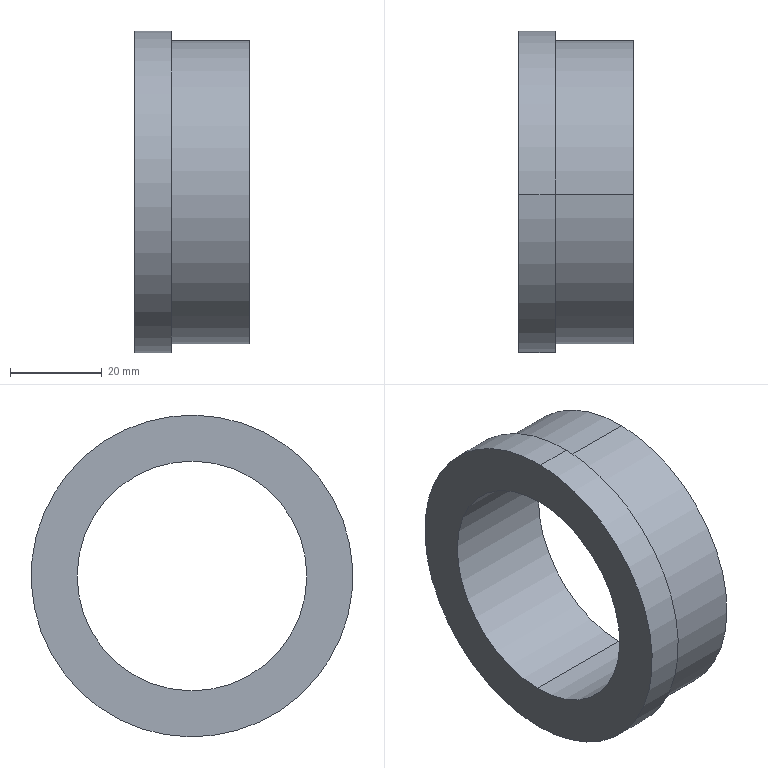Component | SolidWorks | 216InnerTubeAssembly-1_GuideSleeve-1 | 1 solid | 9 faces | box 25 x 70 x 70 mm | volume 39861 mm3 | cylinder 6 | plane 3 | commonest cylinder face diameters 50 x2 66 x2 70 x2 | material Alloy Steel
build123d program:
from build123d import *


with BuildPart() as part:
    # Model → Revolve1 (revolve)
    with BuildSketch(Plane.XY, mode=Mode.PRIVATE) as revolve1_sk:
        Polygon((-25, 35), (-17, 35), (-17, 33), (0, 33), (0, 25), (-25, 25), align=None)
    revolve(revolve1_sk.sketch.rotate(Axis((11.515, 0, 0), (-1, 0, 0)), 90), axis=Axis((11.515, 0, 0), (-1, 0, 0)))


solid = part.part

# Placed as in the assembly
solid = solid.moved(Location((527.091, 0, 0), (0, 0, 0)))
STEP:
#1=COLOUR_RGB('',0.7922,0.8196,0.9333);
#2=FILL_AREA_STYLE_COLOUR('',#1);
#3=FILL_AREA_STYLE('',(#2));
#4=SURFACE_STYLE_FILL_AREA(#3);
#5=SURFACE_SIDE_STYLE('',(#4));
#6=SURFACE_STYLE_USAGE(.BOTH.,#5);
#7=PRESENTATION_STYLE_ASSIGNMENT((#6));
#8=CARTESIAN_POINT('',(19.767,-0.01767,0.9841));
#9=VERTEX_POINT('',#8);
#10=CARTESIAN_POINT('',(19.767,0.01767,-0.9841));
#11=VERTEX_POINT('',#10);
#12=CARTESIAN_POINT('',(19.767,-0.,0.));
#13=DIRECTION('',(1.,0.,-0.));
#14=DIRECTION('',(0.,0.01796,-0.9998));
#15=AXIS2_PLACEMENT_3D('',#12,#13,#14);
#16=CIRCLE('',#15,0.9843);
#17=EDGE_CURVE('',#9,#11,#16,.T.);
#18=ORIENTED_EDGE('',*,*,#17,.F.);
#19=CARTESIAN_POINT('',(20.752,-0.01767,0.9841));
#20=VERTEX_POINT('',#19);
#21=CARTESIAN_POINT('',(21.205,-0.01767,0.9841));
#22=DIRECTION('',(1.,0.,-0.));
#23=VECTOR('',#22,39.37);
#24=LINE('',#21,#23);
#25=EDGE_CURVE('',#9,#20,#24,.T.);
#26=ORIENTED_EDGE('',*,*,#25,.T.);
#27=CARTESIAN_POINT('',(20.752,0.01767,-0.9841));
#28=VERTEX_POINT('',#27);
#29=CARTESIAN_POINT('',(20.752,-0.,0.));
#30=DIRECTION('',(1.,0.,-0.));
#31=DIRECTION('',(0.,0.01796,-0.9998));
#32=AXIS2_PLACEMENT_3D('',#29,#30,#31);
#33=CIRCLE('',#32,0.9843);
#34=EDGE_CURVE('',#20,#28,#33,.T.);
#35=ORIENTED_EDGE('',*,*,#34,.T.);
#36=CARTESIAN_POINT('',(21.205,0.01767,-0.9841));
#37=DIRECTION('',(1.,0.,-0.));
#38=VECTOR('',#37,39.37);
#39=LINE('',#36,#38);
#40=EDGE_CURVE('',#11,#28,#39,.T.);
#41=ORIENTED_EDGE('',*,*,#40,.F.);
#42=EDGE_LOOP('',(#18,#26,#35,#41));
#43=FACE_OUTER_BOUND('',#42,.T.);
#44=CARTESIAN_POINT('',(21.205,-0.,0.));
#45=DIRECTION('',(1.,0.,-0.));
#46=DIRECTION('',(0.,0.01796,-0.9998));
#47=AXIS2_PLACEMENT_3D('',#44,#45,#46);
#48=CYLINDRICAL_SURFACE('',#47,0.9843);
#49=ADVANCED_FACE('',(#43),#48,.F.);
#50=CARTESIAN_POINT('',(20.082,0.02333,-1.299));
#51=VERTEX_POINT('',#50);
#52=CARTESIAN_POINT('',(20.082,-0.02333,1.299));
#53=VERTEX_POINT('',#52);
#54=CARTESIAN_POINT('',(20.082,-0.,0.));
#55=DIRECTION('',(1.,0.,-0.));
#56=DIRECTION('',(0.,0.01796,-0.9998));
#57=AXIS2_PLACEMENT_3D('',#54,#55,#56);
#58=CIRCLE('',#57,1.299);
#59=EDGE_CURVE('',#51,#53,#58,.T.);
#60=ORIENTED_EDGE('',*,*,#59,.T.);
#61=CARTESIAN_POINT('',(20.752,-0.02333,1.299));
#62=VERTEX_POINT('',#61);
#63=CARTESIAN_POINT('',(21.205,-0.02333,1.299));
#64=DIRECTION('',(1.,0.,-0.));
#65=VECTOR('',#64,39.37);
#66=LINE('',#63,#65);
#67=EDGE_CURVE('',#53,#62,#66,.T.);
#68=ORIENTED_EDGE('',*,*,#67,.T.);
#69=CARTESIAN_POINT('',(20.752,0.02333,-1.299));
#70=VERTEX_POINT('',#69);
#71=CARTESIAN_POINT('',(20.752,-0.,0.));
#72=DIRECTION('',(1.,0.,-0.));
#73=DIRECTION('',(0.,0.01796,-0.9998));
#74=AXIS2_PLACEMENT_3D('',#71,#72,#73);
#75=CIRCLE('',#74,1.299);
#76=EDGE_CURVE('',#70,#62,#75,.T.);
#77=ORIENTED_EDGE('',*,*,#76,.F.);
#78=CARTESIAN_POINT('',(21.205,0.02333,-1.299));
#79=DIRECTION('',(1.,0.,-0.));
#80=VECTOR('',#79,39.37);
#81=LINE('',#78,#80);
#82=EDGE_CURVE('',#51,#70,#81,.T.);
#83=ORIENTED_EDGE('',*,*,#82,.F.);
#84=EDGE_LOOP('',(#60,#68,#77,#83));
#85=FACE_OUTER_BOUND('',#84,.T.);
#86=CARTESIAN_POINT('',(21.205,-0.,0.));
#87=DIRECTION('',(1.,0.,-0.));
#88=DIRECTION('',(0.,0.01796,-0.9998));
#89=AXIS2_PLACEMENT_3D('',#86,#87,#88);
#90=CYLINDRICAL_SURFACE('',#89,1.299);
#91=ADVANCED_FACE('',(#85),#90,.T.);
#92=CARTESIAN_POINT('',(19.767,0.02474,-1.378));
#93=VERTEX_POINT('',#92);
#94=CARTESIAN_POINT('',(19.767,-0.02474,1.378));
#95=VERTEX_POINT('',#94);
#96=CARTESIAN_POINT('',(19.767,-0.,0.));
#97=DIRECTION('',(1.,0.,-0.));
#98=DIRECTION('',(0.,0.01796,-0.9998));
#99=AXIS2_PLACEMENT_3D('',#96,#97,#98);
#100=CIRCLE('',#99,1.378);
#101=EDGE_CURVE('',#93,#95,#100,.T.);
#102=ORIENTED_EDGE('',*,*,#101,.T.);
#103=CARTESIAN_POINT('',(20.082,-0.02474,1.378));
#104=VERTEX_POINT('',#103);
#105=CARTESIAN_POINT('',(21.205,-0.02474,1.378));
#106=DIRECTION('',(1.,0.,-0.));
#107=VECTOR('',#106,39.37);
#108=LINE('',#105,#107);
#109=EDGE_CURVE('',#95,#104,#108,.T.);
#110=ORIENTED_EDGE('',*,*,#109,.T.);
#111=CARTESIAN_POINT('',(20.082,0.02474,-1.378));
#112=VERTEX_POINT('',#111);
#113=CARTESIAN_POINT('',(20.082,-0.,0.));
#114=DIRECTION('',(1.,0.,-0.));
#115=DIRECTION('',(0.,0.01796,-0.9998));
#116=AXIS2_PLACEMENT_3D('',#113,#114,#115);
#117=CIRCLE('',#116,1.378);
#118=EDGE_CURVE('',#112,#104,#117,.T.);
#119=ORIENTED_EDGE('',*,*,#118,.F.);
#120=CARTESIAN_POINT('',(21.205,0.02474,-1.378));
#121=DIRECTION('',(1.,0.,-0.));
#122=VECTOR('',#121,39.37);
#123=LINE('',#120,#122);
#124=EDGE_CURVE('',#93,#112,#123,.T.);
#125=ORIENTED_EDGE('',*,*,#124,.F.);
#126=EDGE_LOOP('',(#102,#110,#119,#125));
#127=FACE_OUTER_BOUND('',#126,.T.);
#128=CARTESIAN_POINT('',(21.205,-0.,0.));
#129=DIRECTION('',(1.,0.,-0.));
#130=DIRECTION('',(0.,0.01796,-0.9998));
#131=AXIS2_PLACEMENT_3D('',#128,#129,#130);
#132=CYLINDRICAL_SURFACE('',#131,1.378);
#133=ADVANCED_FACE('',(#127),#132,.T.);
#134=CARTESIAN_POINT('',(19.767,-0.,0.));
#135=DIRECTION('',(1.,0.,-0.));
#136=DIRECTION('',(0.,0.01796,-0.9998));
#137=AXIS2_PLACEMENT_3D('',#134,#135,#136);
#138=CIRCLE('',#137,0.9843);
#139=EDGE_CURVE('',#11,#9,#138,.T.);
#140=ORIENTED_EDGE('',*,*,#139,.T.);
#141=ORIENTED_EDGE('',*,*,#17,.T.);
#142=EDGE_LOOP('',(#140,#141));
#143=FACE_BOUND('',#142,.T.);
#144=ORIENTED_EDGE('',*,*,#101,.F.);
#145=CARTESIAN_POINT('',(19.767,-0.,0.));
#146=DIRECTION('',(1.,0.,-0.));
#147=DIRECTION('',(0.,0.01796,-0.9998));
#148=AXIS2_PLACEMENT_3D('',#145,#146,#147);
#149=CIRCLE('',#148,1.378);
#150=EDGE_CURVE('',#95,#93,#149,.T.);
#151=ORIENTED_EDGE('',*,*,#150,.F.);
#152=EDGE_LOOP('',(#144,#151));
#153=FACE_OUTER_BOUND('',#152,.T.);
#154=CARTESIAN_POINT('',(19.767,1.378,0.02474));
#155=DIRECTION('',(-1.,-0.,0.));
#156=DIRECTION('',(0.,-0.01796,0.9998));
#157=AXIS2_PLACEMENT_3D('',#154,#155,#156);
#158=PLANE('',#157);
#159=ADVANCED_FACE('',(#143,#153),#158,.T.);
#160=ORIENTED_EDGE('',*,*,#109,.F.);
#161=ORIENTED_EDGE('',*,*,#150,.T.);
#162=ORIENTED_EDGE('',*,*,#124,.T.);
#163=CARTESIAN_POINT('',(20.082,-0.,0.));
#164=DIRECTION('',(1.,0.,-0.));
#165=DIRECTION('',(0.,0.01796,-0.9998));
#166=AXIS2_PLACEMENT_3D('',#163,#164,#165);
#167=CIRCLE('',#166,1.378);
#168=EDGE_CURVE('',#104,#112,#167,.T.);
#169=ORIENTED_EDGE('',*,*,#168,.F.);
#170=EDGE_LOOP('',(#160,#161,#162,#169));
#171=FACE_OUTER_BOUND('',#170,.T.);
#172=CARTESIAN_POINT('',(21.205,-0.,0.));
#173=DIRECTION('',(1.,0.,-0.));
#174=DIRECTION('',(0.,0.01796,-0.9998));
#175=AXIS2_PLACEMENT_3D('',#172,#173,#174);
#176=CYLINDRICAL_SURFACE('',#175,1.378);
#177=ADVANCED_FACE('',(#171),#176,.T.);
#178=ORIENTED_EDGE('',*,*,#118,.T.);
#179=ORIENTED_EDGE('',*,*,#168,.T.);
#180=EDGE_LOOP('',(#178,#179));
#181=FACE_OUTER_BOUND('',#180,.T.);
#182=ORIENTED_EDGE('',*,*,#59,.F.);
#183=CARTESIAN_POINT('',(20.082,-0.,0.));
#184=DIRECTION('',(1.,0.,-0.));
#185=DIRECTION('',(0.,0.01796,-0.9998));
#186=AXIS2_PLACEMENT_3D('',#183,#184,#185);
#187=CIRCLE('',#186,1.299);
#188=EDGE_CURVE('',#53,#51,#187,.T.);
#189=ORIENTED_EDGE('',*,*,#188,.F.);
#190=EDGE_LOOP('',(#182,#189));
#191=FACE_BOUND('',#190,.T.);
#192=CARTESIAN_POINT('',(20.082,1.378,0.02474));
#193=DIRECTION('',(1.,0.,-0.));
#194=DIRECTION('',(-0.,0.01796,-0.9998));
#195=AXIS2_PLACEMENT_3D('',#192,#193,#194);
#196=PLANE('',#195);
#197=ADVANCED_FACE('',(#181,#191),#196,.T.);
#198=ORIENTED_EDGE('',*,*,#67,.F.);
#199=ORIENTED_EDGE('',*,*,#188,.T.);
#200=ORIENTED_EDGE('',*,*,#82,.T.);
#201=CARTESIAN_POINT('',(20.752,-0.,0.));
#202=DIRECTION('',(1.,0.,-0.));
#203=DIRECTION('',(0.,0.01796,-0.9998));
#204=AXIS2_PLACEMENT_3D('',#201,#202,#203);
#205=CIRCLE('',#204,1.299);
#206=EDGE_CURVE('',#62,#70,#205,.T.);
#207=ORIENTED_EDGE('',*,*,#206,.F.);
#208=EDGE_LOOP('',(#198,#199,#200,#207));
#209=FACE_OUTER_BOUND('',#208,.T.);
#210=CARTESIAN_POINT('',(21.205,-0.,0.));
#211=DIRECTION('',(1.,0.,-0.));
#212=DIRECTION('',(0.,0.01796,-0.9998));
#213=AXIS2_PLACEMENT_3D('',#210,#211,#212);
#214=CYLINDRICAL_SURFACE('',#213,1.299);
#215=ADVANCED_FACE('',(#209),#214,.T.);
#216=ORIENTED_EDGE('',*,*,#76,.T.);
#217=ORIENTED_EDGE('',*,*,#206,.T.);
#218=EDGE_LOOP('',(#216,#217));
#219=FACE_OUTER_BOUND('',#218,.T.);
#220=CARTESIAN_POINT('',(20.752,-0.,0.));
#221=DIRECTION('',(1.,0.,-0.));
#222=DIRECTION('',(0.,0.01796,-0.9998));
#223=AXIS2_PLACEMENT_3D('',#220,#221,#222);
#224=CIRCLE('',#223,0.9843);
#225=EDGE_CURVE('',#28,#20,#224,.T.);
#226=ORIENTED_EDGE('',*,*,#225,.F.);
#227=ORIENTED_EDGE('',*,*,#34,.F.);
#228=EDGE_LOOP('',(#226,#227));
#229=FACE_BOUND('',#228,.T.);
#230=CARTESIAN_POINT('',(20.752,1.299,0.02333));
#231=DIRECTION('',(1.,0.,-0.));
#232=DIRECTION('',(-0.,0.01796,-0.9998));
#233=AXIS2_PLACEMENT_3D('',#230,#231,#232);
#234=PLANE('',#233);
#235=ADVANCED_FACE('',(#219,#229),#234,.T.);
#236=ORIENTED_EDGE('',*,*,#25,.F.);
#237=ORIENTED_EDGE('',*,*,#139,.F.);
#238=ORIENTED_EDGE('',*,*,#40,.T.);
#239=ORIENTED_EDGE('',*,*,#225,.T.);
#240=EDGE_LOOP('',(#236,#237,#238,#239));
#241=FACE_OUTER_BOUND('',#240,.T.);
#242=CARTESIAN_POINT('',(21.205,-0.,0.));
#243=DIRECTION('',(1.,0.,-0.));
#244=DIRECTION('',(0.,0.01796,-0.9998));
#245=AXIS2_PLACEMENT_3D('',#242,#243,#244);
#246=CYLINDRICAL_SURFACE('',#245,0.9843);
#247=ADVANCED_FACE('',(#241),#246,.F.);
#248=CLOSED_SHELL('',(#49,#91,#133,#159,#177,#197,#215,#235,#247));
#249=MANIFOLD_SOLID_BREP('',#248);
#250=STYLED_ITEM('',(#7),#249);
#251=(LENGTH_UNIT()NAMED_UNIT(*)SI_UNIT($,.METRE.));
#252=LENGTH_MEASURE_WITH_UNIT(LENGTH_MEASURE(0.0254),#251);
#253=DIMENSIONAL_EXPONENTS(1.,0.,0.,0.,0.,0.,0.);
#254=(CONVERSION_BASED_UNIT('',#252)LENGTH_UNIT()NAMED_UNIT(#253));
#255=UNCERTAINTY_MEASURE_WITH_UNIT(LENGTH_MEASURE(0.00001),#254,'','');
#256=(NAMED_UNIT(*)PLANE_ANGLE_UNIT()SI_UNIT($,.RADIAN.));
#257=(NAMED_UNIT(*)SI_UNIT($,.STERADIAN.)SOLID_ANGLE_UNIT());
#258=(GEOMETRIC_REPRESENTATION_CONTEXT(3)GLOBAL_UNCERTAINTY_ASSIGNED_CONTEXT((#255))GLOBAL_UNIT_ASSIGNED_CONTEXT((#254,#256,#257))REPRESENTATION_CONTEXT('',''));
#259=MECHANICAL_DESIGN_GEOMETRIC_PRESENTATION_REPRESENTATION('',(#250),#258);
#260=CARTESIAN_POINT('',(0.,0.,0.));
#261=DIRECTION('',(0.,0.,1.));
#262=DIRECTION('',(1.,0.,0.));
#263=AXIS2_PLACEMENT_3D('',#260,#261,#262);
#264=(LENGTH_UNIT()NAMED_UNIT(*)SI_UNIT($,.METRE.));
#265=LENGTH_MEASURE_WITH_UNIT(LENGTH_MEASURE(0.0254),#264);
#266=DIMENSIONAL_EXPONENTS(1.,0.,0.,0.,0.,0.,0.);
#267=(CONVERSION_BASED_UNIT('',#265)LENGTH_UNIT()NAMED_UNIT(#266));
#268=UNCERTAINTY_MEASURE_WITH_UNIT(LENGTH_MEASURE(0.00001),#267,'','');
#269=(NAMED_UNIT(*)PLANE_ANGLE_UNIT()SI_UNIT($,.RADIAN.));
#270=(NAMED_UNIT(*)SI_UNIT($,.STERADIAN.)SOLID_ANGLE_UNIT());
#271=(GEOMETRIC_REPRESENTATION_CONTEXT(3)GLOBAL_UNCERTAINTY_ASSIGNED_CONTEXT((#268))GLOBAL_UNIT_ASSIGNED_CONTEXT((#267,#269,#270))REPRESENTATION_CONTEXT('',''));
#272=ADVANCED_BREP_SHAPE_REPRESENTATION('',(#249,#263),#271);
#273=PRESENTATION_LAYER_ASSIGNMENT('','',(#250));